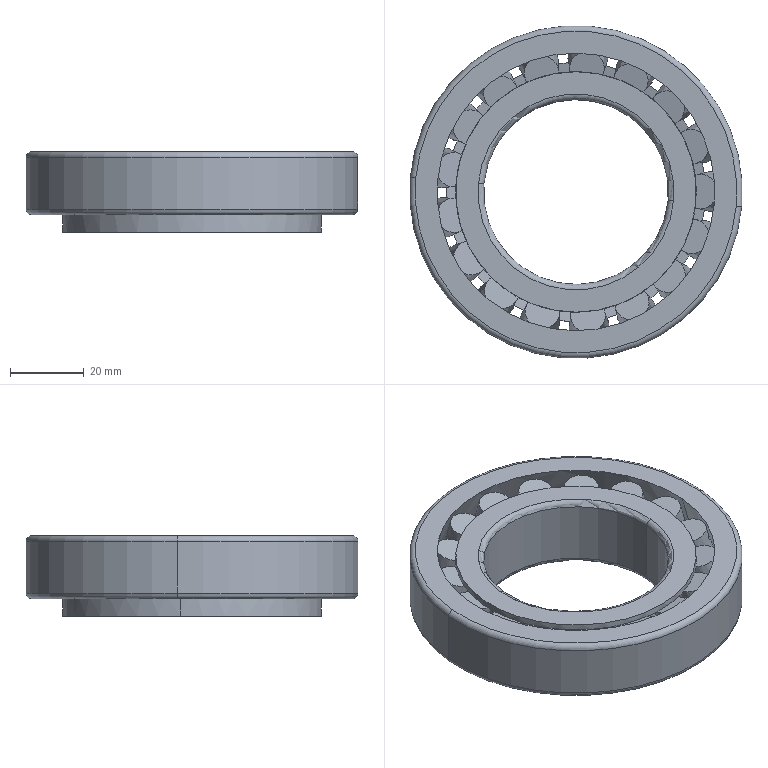Component | SolidWorks | GB_T297-94TaperedRollerBearing30210-0717-1 | 1 solid | 144 faces | volume 64245 mm3 | cone 90 | plane 38 | torus 8 | cylinder 8 | commonest cylinder face diameters 90 x2 50 x2 65.047 x2 70.062 x2